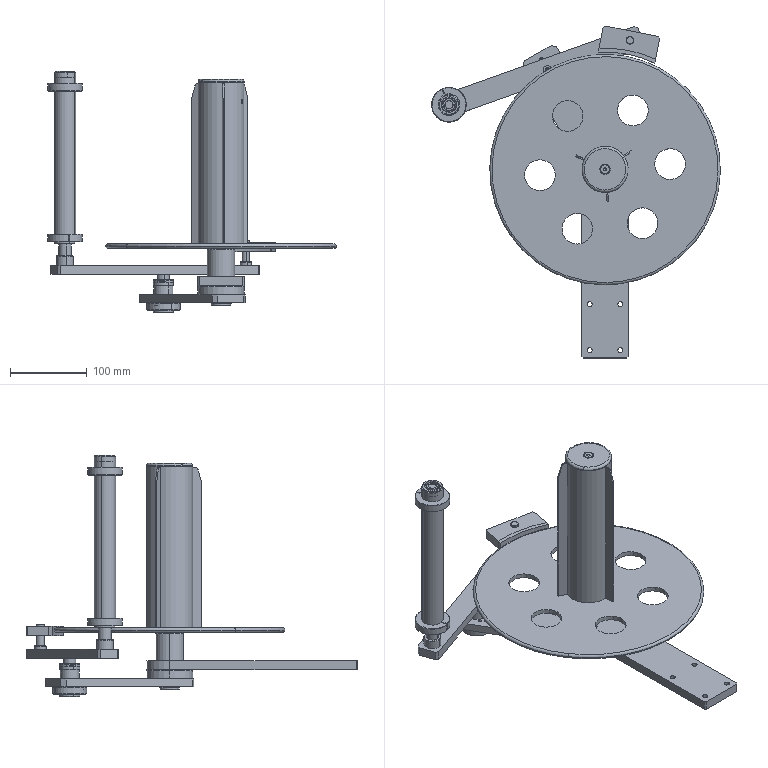Assembly | SolidWorks | mm | 39 component files | 40 solids | 1339 faces | box 375.57 x 431.83 x 314 mm | volume 1536766 mm3 | plane 378 | cylinder 345 | torus 332 | sphere 156 | cone 128 | commonest cylinder face diameters 10 x31 20.667 x24 15.333 x24 6.6 x20 11 x18 5.5 x18 1.6 x18 3 x18
Bill of materials:
circlips for shaft--type a large gb | 1 |  | Thin flat split ring with a radial gap; two widened lugs at the gap ends, each with a small round through hole. Shape is consistent with an external retaining-ring style clip.
deep groove ball bearings gb | 6 |  | Radial ball bearing-like assembly body: outer ring, inner ring with central bore, and a single row of spherical balls between them; no cage or seals visible.
hexagon socket countersunk head screws gb | 4 |  | Solid axisymmetric part: a cylindrical post with a chamfered top end rising from a conical skirt that ends in a short cylindrical base rim.
hexagon socket head cap screws gb | 9 |  | Cap-screw-like solid: a cylindrical head with a hexagonal socket recess, on a plain cylindrical shank with a chamfered end.
JYTBJ-HeaderBrakeAxis | 1 | AISI 1045 Steel, Cold Drawn | Headed cylindrical pin-like part: a larger cylindrical head with a small central hole in its end face, and a long smooth shank with a narrow circumferential groove near the far end.
JYTBJ-HeaderBrakeLever | 1 |  | Long, thin, flat rectangular bar with chamfered corners and three main round through holes: one near each end and one at the middle. There is also a smaller extra hole near one end.
JYTBJ-HeaderPlate | 1 |  | Thin flat circular disc with six large round holes evenly spaced on a ring, a small central round hole, and three small holes around the center.
JYTBJ-HeaderPlateAxisBarrelCover | 1 | 5052-H32 | Thin circular disc with a rounded outer edge on one face and a single central countersunk through hole.
JYTBJ-HeaderPlateBrakeAxis | 1 |  | Stepped solid cylindrical pin: a short larger-diameter collar at one end and a longer smaller-diameter shaft, with chamfers on the end edges.
JYTBJ-HeaderPlateBrakePad | 1 |  | Thick block shaped like an arc segment: one long side is concave-curved, the opposite side straight, the ends are angled with small corner chamfers, and there is one round through hole.
JYTBJ-HeaderPlateClampBlock | 3 |  | Straight extruded bar with a T-shaped cross-section; one end is tapered or angled off.
JYTBJ-HeaderPlateFlangeSeatA | 1 |  | Flanged tubular bushing-like part: a cylindrical sleeve with a through bore and a round flange near one end, the flange having three evenly spaced through holes. The sleeve continues a short distance past the flange.
JYTBJ-HeaderPlateFlangeSeatB | 1 |  | Flanged cylindrical bushing: a round flange with three through holes and a hollow cylindrical boss standing up from it.
JYTBJ-HeaderPlateRotatingAxis | 1 |  | Long, thin cylindrical rod with a small, thin collar at one end and a small axial hole or recess at the other end.
JYTBJ-HeaderPlateRotatingAxisBarrel | 1 |  | Solid cylinder with a central axial through bore, three rectangular axial through cavities spaced around the bore, and narrow slits running the full length from each cavity to the outer surface.
JYTBJ-HeaderPlateSupportFrame | 1 |  | Flat, long plate with one semicircular end and one squared end. It has a large circular hole near the rounded end, a few small holes around that hole, and four small holes in a rectangular pattern near the other end.
JYTBJ-HeaderPlateSupportFrameA | 1 |  | Flat rectangular plate with chamfered corners and two circular through holes of different sizes, one near each end. Each large hole has three small holes around it.
JYTBJ-HeaderRoller | 1 |  | Long, straight tube with a plain cylindrical outside and a concentric through bore.
JYTBJ-HeaderRollerAxis | 1 |  | Long, thin solid pin with a two-step enlarged section at one end.
JYTBJ-LabelLimitSleeve | 2 |  | Thick, flat ring with a single narrow radial split through its full section.
Mates:
1. concentric | JYTBJ-HeaderPlateSupportFrame-1 face at (3.373, 96.878, 6) dir (0, 0, -1) r 18.05 | JYTBJ-HeaderPlateFlangeSeatA-1 face at (3.373, 96.878, 42) dir (0, 0, 1) r 18
2. concentric | JYTBJ-HeaderPlateSupportFrame-1 face at (27.373, 96.878, 6) dir (0, 0, 1) r 5 | JYTBJ-HeaderPlateFlangeSeatA-1 face at (27.373, 96.878, -6) dir (0, 0, 1) r 2.75
3. coincident | JYTBJ-HeaderPlateFlangeSeatA-1 face at (3.373, 78.878, -6) dir (0, 0, 1) | JYTBJ-HeaderPlateSupportFrame-1 face at (3.373, 96.878, -6) dir (0, 0, -1)
4. concentric | JYTBJ-HeaderPlateFlangeSeatA-1 face at (3.373, 96.878, 42) dir (0, 0, 1) r 18 | JYTBJ-HeaderPlateSupportFrameA-1 face at (3.373, 96.878, -18) dir (0, 0, -1) r 18.05
5. coincident | JYTBJ-HeaderPlateFlangeSeatA-1 face at (3.373, 66.878, -18) dir (0, 0, -1) | JYTBJ-HeaderPlateSupportFrameA-1 face at (-5.777, 62.727, -18) dir (0, 0, 1)
6. concentric | JYTBJ-HeaderPlateSupportFrameA-1 face at (-71.627, 226.781, -18) dir (0, 0, -1) r 12.5 | JYTBJ-HeaderPlateFlangeSeatB-1 face at (-71.627, 226.781, -34.485) dir (0, 0, -1) r 12.5
7. concentric | JYTBJ-HeaderPlateSupportFrameA-1 face at (-79.627, 240.638, -18) dir (0, 0, 1) r 2.1 | JYTBJ-HeaderPlateFlangeSeatB-1 face at (-79.627, 240.638, -38) dir (0, 0, -1) r 5
8. coincident | JYTBJ-HeaderPlateSupportFrameA-1 face at (-5.777, 62.727, -28) dir (0, 0, -1) | JYTBJ-HeaderPlateFlangeSeatB-1 face at (-82.452, 220.531, -28) dir (0, 0, 1)
9. concentric | JYTBJ-HeaderBrakeAxis-1 face at (-71.627, 226.781, 11) dir (0, 0, 1) r 2.5 | JYTBJ-HeaderBrakeLever-1 face at (-71.627, 226.781, 21) dir (0, 0, 1) r 5.5
10. concentric | JYTBJ-HeaderBrakeLever-1 face at (-71.627, 226.781, 21) dir (0, 0, 1) r 5.5 | JYTBJ-HeaderBrakeAxis-1 face at (-71.627, 226.781, 11) dir (0, 0, 1) r 2.5
11. coincident | JYTBJ-HeaderBrakeLever-1 face at (-71.627, 226.781, 11) dir (0, 0, -1) | JYTBJ-HeaderBrakeAxis-1 face at (-71.627, 226.781, 11) dir (0, 0, 1)
12. concentric | JYTBJ-HeaderPlateBrakeAxis-1 face at (35.724, 265.147, 18) dir (0, 0, -1) r 7.5 | JYTBJ-HeaderBrakeLever-1 face at (35.724, 265.147, 9) dir (0, 0, -1) r 5.5
13. coincident | JYTBJ-HeaderBrakeLever-1 face at (35.724, 265.147, 18) dir (0, 0, 1) | JYTBJ-HeaderPlateBrakeAxis-1 face at (35.724, 265.147, 18) dir (0, 0, -1)
14. concentric | JYTBJ-HeaderPlateFlangeSeatA-1 face at (3.373, 96.878, 42) dir (0, 0, 1) r 16 | deep groove ball bearings gb-1 face at (3.373, 96.878, -16.289) dir (0, 0, 1) r 13
15. coincident | JYTBJ-HeaderPlateFlangeSeatA-1 face at (3.373, 80.878, -21) dir (0, 0, -1) | deep groove ball bearings gb-1 face at (3.373, 109.878, -21) dir (0, 0, 1)
16. coincident | deep groove ball bearings gb-1 face at (3.373, 101.878, -29) dir (0, 0, -1) | JYTBJ-HeaderPlateRotatingAxis-1 face at (3.373, 96.878, -29) dir (0, 0, 1)
17. concentric | JYTBJ-HeaderPlateRotatingAxis-1 face at (3.373, 96.878, -29) dir (0, 0, 1) r 10 | JYTBJ-HeaderPlateRotatingAxisBarrel-1 face at (3.373, 96.878, 48.5) dir (0, 0, 1) r 30
18. concentric | JYTBJ-HeaderPlateRotatingAxisBarrel-1 face at (3.373, 96.878, 42) dir (0, 0, 1) r 13 | JYTBJ-HeaderPlate-1 face at (3.373, 96.878, 48.5) dir (0, 0, -1) r 13.25
19. concentric | JYTBJ-HeaderPlateRotatingAxisBarrel-1 face at (1.675, 116.805, 48.5) dir (0, 0, -1) r 3 | JYTBJ-HeaderPlate-1 face at (1.675, 116.805, 42.5) dir (0, 0, -1) r 3.3
20. coincident | JYTBJ-HeaderPlateRotatingAxisBarrel-1 face at (3.373, 96.878, 48.5) dir (0, 0, -1) | JYTBJ-HeaderPlate-1 face at (3.373, 96.878, 48.5) dir (0, 0, 1)
21. concentric | JYTBJ-HeaderBrakeLever-1 face at (-199.694, 181.012, 18) dir (0, 0, 1) r 11 | JYTBJ-HeaderRollerBody-1/JYTBJ-HeaderRoller-1 face at (-199.694, 181.012, 271) dir (0, 0, -1) r 14
22. coincident | JYTBJ-HeaderBrakeLever-1 face at (-199.694, 181.012, 18) dir (0, 0, 1) | JYTBJ-HeaderRollerBody-1/JYTBJ-HeaderRollerAxis-1 face at (-199.694, 181.012, 18) dir (0, 0, -1)
23. concentric | JYTBJ-HeaderPlateFlangeSeatB-1 face at (-71.627, 226.781, -34.485) dir (0, 0, -1) r 12.5 | JYTBJ-HeaderBrakeAxis-1 face at (-71.627, 226.781, -1) dir (0, 0, -1) r 6
24. coincident | JYTBJ-HeaderBrakeAxis-1 face at (-71.627, 226.781, -1) dir (0, 0, -1) | JYTBJ-HeaderPlateFlangeSeatB-1 face at (-80.72, 221.531, -1) dir (0, 0, 1)
25. concentric | JYTBJ-HeaderPlateBrakeAxis-1 face at (35.724, 265.147, 18) dir (0, 0, -1) r 5 | JYTBJ-HeaderPlateBrakePad-1 face at (35.724, 265.147, 38.5) dir (0, 0, 1) r 5
26. coincident | JYTBJ-HeaderPlateRotatingAxisBarrel-1 face at (-17.618, 113.35, 258.5) dir (0.9054, -0.4246, 0) | JYTBJ-HeaderPlateClampBlock-1 face at (-18.043, 112.445, 48.5) dir (-0.9054, 0.4246, 0)
27. coincident | JYTBJ-HeaderPlateRotatingAxisBarrel-1 face at (-29.844, 111.353, 258.5) dir (0.4246, 0.9054, 0) | JYTBJ-HeaderPlateClampBlock-1 face at (-20.591, 107.013, 48.5) dir (-0.4246, -0.9054, 0)
28. coincident | JYTBJ-HeaderPlate-1 face at (3.373, 96.878, 48.5) dir (0, 0, 1) | JYTBJ-HeaderPlateClampBlock-1 face at (-34.227, 115.618, 48.5) dir (0, 0, -1)
29. coincident | JYTBJ-HeaderPlateRotatingAxisBarrel-1 face at (7.446, 60.873, 258.5) dir (-0.9964, -0.08494, 0) | JYTBJ-HeaderPlateClampBlock-2 face at (6.578, 71.057, 48.5) dir (0.9964, 0.08494, 0)
30. coincident | JYTBJ-HeaderPlateRotatingAxisBarrel-1 face at (-0.3965, 70.462, 258.5) dir (-0.08494, 0.9964, 0) | JYTBJ-HeaderPlateClampBlock-2 face at (0.5999, 70.547, 48.5) dir (0.08494, -0.9964, 0)
31. coincident | JYTBJ-HeaderPlate-1 face at (3.373, 96.878, 48.5) dir (0, 0, 1) | JYTBJ-HeaderPlateClampBlock-2 face at (5.944, 54.944, 48.5) dir (0, 0, -1)
32. coincident | JYTBJ-HeaderPlateRotatingAxisBarrel-1 face at (24.133, 112.564, 258.5) dir (-0.8204, -0.5718, 0) | JYTBJ-HeaderPlateClampBlock-3 face at (21.846, 115.845, 48.5) dir (0.8204, 0.5718, 0)
33. coincident | JYTBJ-HeaderPlateRotatingAxisBarrel-1 face at (32.518, 118.407, 258.5) dir (0.5718, -0.8204, 0) | JYTBJ-HeaderPlateClampBlock-3 face at (24.133, 112.564, 48.5) dir (-0.5718, 0.8204, 0)
34. coincident | JYTBJ-HeaderPlate-1 face at (3.373, 96.878, 48.5) dir (0, 0, 1) | JYTBJ-HeaderPlateClampBlock-3 face at (38.403, 120.071, 48.5) dir (0, 0, -1)
35. concentric | JYTBJ-HeaderPlateRotatingAxis-1 face at (3.373, 96.878, 201) dir (0, 0, 1) r 2.5 | JYTBJ-HeaderPlateAxisBarrelCover-1 face at (3.373, 96.878, 262.5) dir (0, 0, 1) r 3.3
36. concentric | JYTBJ-HeaderBrakeAxis-1 face at (-71.627, 226.781, -1) dir (0, 0, -1) r 6 | circlips for shaft--type a large gb-1 face at (-71.627, 226.781, -38) dir (0, 0, -1) r 4.65
37. coincident | JYTBJ-HeaderBrakeAxis-1 face at (-70.401, 221.42, -38) dir (0, 0, -1) | circlips for shaft--type a large gb-1 face at (-71.627, 226.781, -38) dir (0, 0, 1)
38. coincident | hexagon socket head cap screws gb-1 face at (-8.627, 117.662, 0.3) dir (0, 0, -1) | hexagon socket head cap screws gb-2 face at (-8.627, 76.093, 0.3) dir (0, 0, -1)
39. coincident | hexagon socket head cap screws gb-2 face at (-8.627, 76.093, 0.3) dir (0, 0, -1) | hexagon socket head cap screws gb-3 face at (27.373, 96.878, 0.3) dir (0, 0, -1)
40. coincident | JYTBJ-HeaderPlateSupportFrame-1 face at (30.123, 96.878, 0.3) dir (0, 0, 1) | hexagon socket head cap screws gb-3 face at (27.373, 96.878, 0.3) dir (0, 0, -1)
41. concentric | JYTBJ-HeaderPlateFlangeSeatB-1 face at (-79.627, 240.638, -38) dir (0, 0, -1) r 5 | hexagon socket head cap screws gb-4 face at (-79.627, 240.638, -26.3) dir (0, 0, -1) r 0.8
42. concentric | JYTBJ-HeaderPlateFlangeSeatB-1 face at (-79.627, 212.925, -38) dir (0, 0, -1) r 5 | hexagon socket head cap screws gb-5 face at (-79.627, 212.925, -26.3) dir (0, 0, -1) r 0.8
43. concentric | JYTBJ-HeaderPlateFlangeSeatB-1 face at (-55.627, 226.781, -38) dir (0, 0, -1) r 5 | hexagon socket head cap screws gb-6 face at (-55.627, 226.781, -26.3) dir (0, 0, -1) r 0.8
44. coincident | hexagon socket head cap screws gb-4 face at (-79.627, 240.638, -32.3) dir (0, 0, 1) | hexagon socket head cap screws gb-5 face at (-79.627, 212.925, -32.3) dir (0, 0, 1)
45. coincident | hexagon socket head cap screws gb-5 face at (-79.627, 212.925, -32.3) dir (0, 0, 1) | hexagon socket head cap screws gb-6 face at (-55.627, 226.781, -32.3) dir (0, 0, 1)
46. coincident | JYTBJ-HeaderPlateFlangeSeatB-1 face at (-58.008, 225.406, -32.3) dir (0, 0, -1) | hexagon socket head cap screws gb-6 face at (-55.627, 226.781, -32.3) dir (0, 0, 1)
47. concentric | JYTBJ-HeaderBrakeLever-1 face at (35.724, 265.147, 9) dir (0, 0, -1) r 5.5 | hexagon socket head cap screws gb-7 face at (35.724, 265.147, 21.8) dir (0, 0, -1) r 0.8
48. concentric | JYTBJ-HeaderBrakeLever-1 face at (-199.694, 181.012, 9) dir (0, 0, -1) r 5.5 | hexagon socket head cap screws gb-8 face at (-199.694, 181.012, 21.8) dir (0, 0, -1) r 0.8
49. coincident | JYTBJ-HeaderBrakeLever-1 face at (-202.801, 179.902, 15.8) dir (0, 0, -1) | hexagon socket head cap screws gb-8 face at (-199.694, 181.012, 15.8) dir (0, 0, 1)
50. coincident | JYTBJ-HeaderBrakeLever-1 face at (32.616, 264.036, 15.8) dir (0, 0, -1) | hexagon socket head cap screws gb-7 face at (35.724, 265.147, 15.8) dir (0, 0, 1)
51. concentric | JYTBJ-HeaderBrakeLever-1 face at (-71.627, 226.781, 21) dir (0, 0, 1) r 5.5 | hexagon socket head cap screws gb-11 face at (-71.627, 226.781, 8.2) dir (0, 0, 1) r 0.8
52. coincident | JYTBJ-HeaderBrakeLever-1 face at (-74.452, 225.772, 14.2) dir (0, 0, 1) | hexagon socket head cap screws gb-11 face at (-71.627, 226.781, 14.2) dir (0, 0, -1)
53. concentric | JYTBJ-HeaderPlate-1 face at (21.481, 88.385, 42.5) dir (0, 0, -1) r 3.3 | hexagon socket countersunk head screws gb-1 face at (21.481, 88.385, 41.913) dir (0, 0, -1) r 3
54. concentric | JYTBJ-HeaderPlate-1 face at (1.675, 116.805, 42.5) dir (0, 0, -1) r 3.3 | hexagon socket countersunk head screws gb-3 face at (1.675, 116.805, 41.913) dir (0, 0, -1) r 3
55. concentric | JYTBJ-HeaderPlate-1 face at (-13.035, 85.443, 42.5) dir (0, 0, -1) r 3.3 | hexagon socket countersunk head screws gb-2 face at (-13.035, 85.443, 41.913) dir (0, 0, -1) r 3
56. coincident | hexagon socket countersunk head screws gb-1 face at (21.481, 88.385, 42.5) dir (0, 0, -1) | hexagon socket countersunk head screws gb-3 face at (1.675, 116.805, 42.5) dir (0, 0, -1)
57. coincident | hexagon socket countersunk head screws gb-2 face at (-13.035, 85.443, 42.5) dir (0, 0, -1) | hexagon socket countersunk head screws gb-3 face at (1.675, 116.805, 42.5) dir (0, 0, -1)
58. coincident | JYTBJ-HeaderPlate-1 face at (3.373, 96.878, 42.5) dir (0, 0, -1) | hexagon socket countersunk head screws gb-1 face at (21.481, 88.385, 42.5) dir (0, 0, -1)
59. concentric | JYTBJ-HeaderPlateRotatingAxis-1 face at (3.373, 96.878, 201) dir (0, 0, 1) r 2.5 | hexagon socket countersunk head screws gb-4 face at (3.373, 96.878, 263.087) dir (0, 0, 1) r 3
60. coincident | JYTBJ-HeaderPlateAxisBarrelCover-1 face at (3.373, 96.878, 262.5) dir (0, 0, 1) | hexagon socket countersunk head screws gb-4 face at (3.373, 96.878, 262.5) dir (0, 0, 1)
61. coincident | JYTBJ-HeaderPlateFlangeSeatA-1 face at (3.373, 80.878, 42) dir (0, 0, 1) | JYTBJ-HeaderPlateRotatingAxisBarrel-1 face at (3.373, 96.878, 42) dir (0, 0, -1)
62. coincident | JYTBJ-HeaderPlateRotatingAxisBarrel-1 face at (3.373, 96.878, 258.5) dir (0, 0, 1) | JYTBJ-HeaderPlateAxisBarrelCover-1 face at (3.373, 96.878, 258.5) dir (0, 0, -1)
63. distance | JYTBJ-HeaderPlateBrakePad-1 face at (3.562, 99.851, 50.5) dir (0, 0, 1) | JYTBJ-HeaderPlate-1 face at (3.373, 96.878, 48.5) dir (0, 0, 1)
64. concentric | JYTBJ-HeaderPlateFlangeSeatA-1 face at (-8.627, 76.093, -6) dir (0, 0, 1) r 2.75 | JYTBJ-HeaderPlateSupportFrameA-1 face at (-8.627, 76.093, -18) dir (0, 0, 1) r 2.1
65. concentric | JYTBJ-HeaderBrakeAxis-1 face at (-71.627, 226.781, 11) dir (0, 0, -1) r 8 | deep groove ball bearings gb-2 face at (-71.627, 226.781, -10.711) dir (0, 0, -1) r 13
66. coincident | JYTBJ-HeaderPlateFlangeSeatB-1 face at (-78.555, 222.781, -6) dir (0, 0, 1) | deep groove ball bearings gb-2 face at (-66.647, 214.773, -6) dir (0, 0, -1)
67. concentric | JYTBJ-HeaderPlateFlangeSeatB-1 face at (-71.627, 226.781, -34.485) dir (0, 0, -1) r 10.5 | deep groove ball bearings gb-3 face at (-71.627, 226.781, -45.711) dir (0, 0, -1) r 13
68. coincident | JYTBJ-HeaderPlateFlangeSeatB-1 face at (-80.72, 221.531, -33) dir (0, 0, -1) | deep groove ball bearings gb-3 face at (-66.647, 214.773, -33) dir (0, 0, 1)
69. concentric | JYTBJ-HeaderPlateRotatingAxis-1 face at (3.373, 96.878, -29) dir (0, 0, 1) r 10 | deep groove ball bearings gb-5 face at (3.373, 96.878, 47.711) dir (0, 0, 1) r 13
70. coincident | JYTBJ-HeaderPlateFlangeSeatA-1 face at (3.373, 83.878, 35) dir (0, 0, 1) | deep groove ball bearings gb-5 face at (5.289, 92.259, 35) dir (0, 0, -1)
71. concentric | JYTBJ-HeaderRollerAxis-1 face at (149.057, -3.306, 0) dir (-1, 0, 0) r 6 | deep groove ball bearings gb-2 face at (-70.654, -3.306, 0) dir (-1, 0, 0) r 13
72. coincident | JYTBJ-HeaderRollerAxis-1 face at (-65.943, -3.306, 0) dir (1, 0, 0) | deep groove ball bearings gb-2 face at (-65.943, 4.195, 1.587) dir (-1, 0, 0)
73. coincident | JYTBJ-HeaderRoller-1 face at (-57.943, -3.306, 0) dir (-1, 0, 0) | deep groove ball bearings gb-2 face at (-57.943, 9.413, 2.691) dir (1, 0, 0)
74. concentric | JYTBJ-HeaderRollerAxis-1 face at (149.057, -3.306, 0) dir (-1, 0, 0) r 6 | JYTBJ-HeaderRoller-1 face at (156.057, -3.306, 0) dir (-1, 0, 0) r 14
75. coincident | JYTBJ-HeaderRoller-1 face at (150.057, -3.306, 0) dir (1, 0, 0) | deep groove ball bearings gb-3 face at (150.057, 4.361, 0) dir (-1, 0, 0)
76. concentric | JYTBJ-HeaderRollerAxis-1 face at (149.057, -3.306, 0) dir (-1, 0, 0) r 6 | deep groove ball bearings gb-3 face at (147.085, -3.306, 0) dir (-1, 0, 0) r 5
77. concentric | JYTBJ-HeaderRoller-1 face at (156.057, -3.306, 0) dir (-1, 0, 0) r 14 | JYTBJ-LabelLimitSleeve-1 face at (-53.943, -3.306, 0) dir (-1, 0, 0) r 14
78. coincident | JYTBJ-HeaderRoller-1 face at (-63.943, -3.306, 0) dir (-1, 0, 0) | JYTBJ-LabelLimitSleeve-1 face at (-63.943, -3.306, 0) dir (-1, 0, 0)
79. concentric | JYTBJ-HeaderRoller-1 face at (156.057, -3.306, 0) dir (-1, 0, 0) r 14 | JYTBJ-LabelLimitSleeve-2 face at (132.386, -3.306, 0) dir (1, 0, 0) r 14